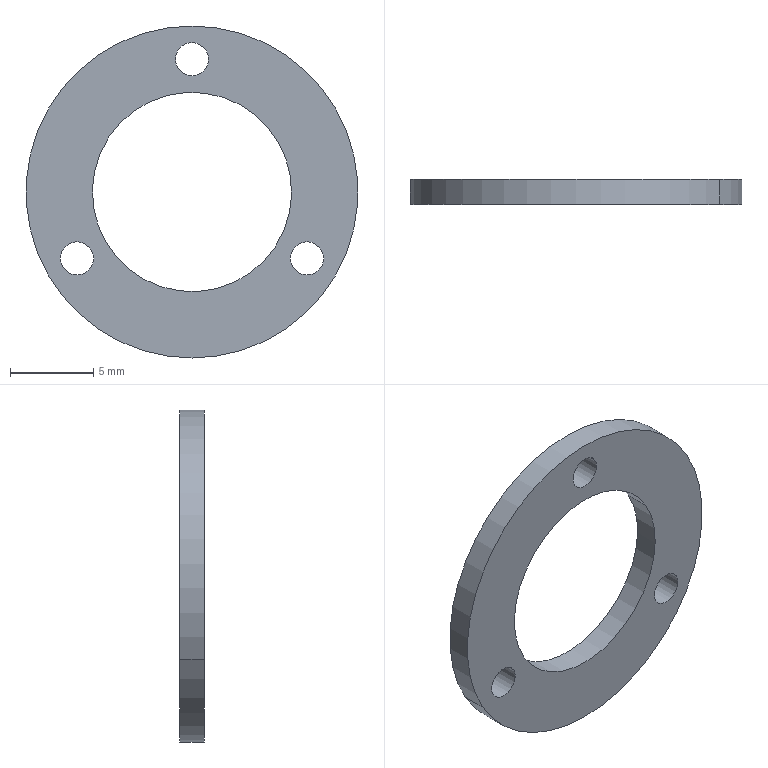Component | SolidWorks | NozzleGasket2-1 | 1 solid | 12 faces | box 20 x 1.5 x 20 mm | volume 287 mm3 | cylinder 10 | plane 2 | commonest cylinder face diameters 2 x6 12 x2 20 x2
build123d program:
from build123d import *

# Parameters (mm, degrees)
SKETCH1_R           = 10
SKETCH1_R_2         = 1
SKETCH1_R_3         = 6
BOSS_EXTRUDE1_DEPTH = 1.5


with BuildPart() as part:
    # Sketch1 → Boss-Extrude1 (new body)
    with BuildSketch(Plane(origin=(0, 0, 0), x_dir=(1, 0, 0), z_dir=(0, 1, 0))):
        with Locations(Location((0, 0, 0), (0, 0, 270))):
            Circle(SKETCH1_R)
        with Locations(Location((0, 8, 0), (0, 0, 270))):
            Circle(SKETCH1_R_2, mode=Mode.SUBTRACT)
        with Locations(Location((6.928, -4, 0), (0, 0, 270))):
            Circle(SKETCH1_R_2, mode=Mode.SUBTRACT)
        with Locations(Location((-6.928, -4, 0), (0, 0, 270))):
            Circle(SKETCH1_R_2, mode=Mode.SUBTRACT)
        with Locations(Location((0, 0, 0), (0, 0, 270))):
            Circle(SKETCH1_R_3, mode=Mode.SUBTRACT)
    extrude(amount=BOSS_EXTRUDE1_DEPTH)


solid = part.part

# Placed as in the assembly
solid = solid.moved(Location((-5.981, -106.494, 160), (180, 0, 0)))
STEP:
#1=COLOUR_RGB('',0.7922,0.8196,0.9333);
#2=FILL_AREA_STYLE_COLOUR('',#1);
#3=FILL_AREA_STYLE('',(#2));
#4=SURFACE_STYLE_FILL_AREA(#3);
#5=SURFACE_SIDE_STYLE('',(#4));
#6=SURFACE_STYLE_USAGE(.BOTH.,#5);
#7=PRESENTATION_STYLE_ASSIGNMENT((#6));
#8=CARTESIAN_POINT('',(-0.2696,-4.193,6.594));
#9=VERTEX_POINT('',#8);
#10=CARTESIAN_POINT('',(-0.2014,-4.193,6.634));
#11=VERTEX_POINT('',#10);
#12=CARTESIAN_POINT('',(-0.2355,-4.193,6.614));
#13=DIRECTION('',(-0.,1.,0.));
#14=DIRECTION('',(0.866,0.,0.5));
#15=AXIS2_PLACEMENT_3D('',#12,#13,#14);
#16=CIRCLE('',#15,0.03937);
#17=EDGE_CURVE('',#9,#11,#16,.T.);
#18=ORIENTED_EDGE('',*,*,#17,.T.);
#19=CARTESIAN_POINT('',(-0.2014,-4.252,6.634));
#20=VERTEX_POINT('',#19);
#21=CARTESIAN_POINT('',(-0.2014,-4.193,6.634));
#22=DIRECTION('',(0.,-1.,-0.));
#23=VECTOR('',#22,39.37);
#24=LINE('',#21,#23);
#25=EDGE_CURVE('',#11,#20,#24,.T.);
#26=ORIENTED_EDGE('',*,*,#25,.T.);
#27=CARTESIAN_POINT('',(-0.2696,-4.252,6.594));
#28=VERTEX_POINT('',#27);
#29=CARTESIAN_POINT('',(-0.2355,-4.252,6.614));
#30=DIRECTION('',(-0.,1.,0.));
#31=DIRECTION('',(0.866,0.,0.5));
#32=AXIS2_PLACEMENT_3D('',#29,#30,#31);
#33=CIRCLE('',#32,0.03937);
#34=EDGE_CURVE('',#28,#20,#33,.T.);
#35=ORIENTED_EDGE('',*,*,#34,.F.);
#36=CARTESIAN_POINT('',(-0.2696,-4.193,6.594));
#37=DIRECTION('',(0.,-1.,-0.));
#38=VECTOR('',#37,39.37);
#39=LINE('',#36,#38);
#40=EDGE_CURVE('',#9,#28,#39,.T.);
#41=ORIENTED_EDGE('',*,*,#40,.F.);
#42=EDGE_LOOP('',(#18,#26,#35,#41));
#43=FACE_OUTER_BOUND('',#42,.T.);
#44=CARTESIAN_POINT('',(-0.2355,-4.193,6.614));
#45=DIRECTION('',(0.,-1.,-0.));
#46=DIRECTION('',(-0.866,0.,-0.5));
#47=AXIS2_PLACEMENT_3D('',#44,#45,#46);
#48=CYLINDRICAL_SURFACE('',#47,0.03937);
#49=ADVANCED_FACE('',(#43),#48,.F.);
#50=CARTESIAN_POINT('',(0.0032,-4.193,6.122));
#51=VERTEX_POINT('',#50);
#52=CARTESIAN_POINT('',(0.07139,-4.193,6.161));
#53=VERTEX_POINT('',#52);
#54=CARTESIAN_POINT('',(0.0373,-4.193,6.142));
#55=DIRECTION('',(-0.,1.,0.));
#56=DIRECTION('',(0.866,0.,0.5));
#57=AXIS2_PLACEMENT_3D('',#54,#55,#56);
#58=CIRCLE('',#57,0.03937);
#59=EDGE_CURVE('',#51,#53,#58,.T.);
#60=ORIENTED_EDGE('',*,*,#59,.T.);
#61=CARTESIAN_POINT('',(0.07139,-4.252,6.161));
#62=VERTEX_POINT('',#61);
#63=CARTESIAN_POINT('',(0.07139,-4.193,6.161));
#64=DIRECTION('',(0.,-1.,-0.));
#65=VECTOR('',#64,39.37);
#66=LINE('',#63,#65);
#67=EDGE_CURVE('',#53,#62,#66,.T.);
#68=ORIENTED_EDGE('',*,*,#67,.T.);
#69=CARTESIAN_POINT('',(0.0032,-4.252,6.122));
#70=VERTEX_POINT('',#69);
#71=CARTESIAN_POINT('',(0.0373,-4.252,6.142));
#72=DIRECTION('',(-0.,1.,0.));
#73=DIRECTION('',(0.866,0.,0.5));
#74=AXIS2_PLACEMENT_3D('',#71,#72,#73);
#75=CIRCLE('',#74,0.03937);
#76=EDGE_CURVE('',#70,#62,#75,.T.);
#77=ORIENTED_EDGE('',*,*,#76,.F.);
#78=CARTESIAN_POINT('',(0.0032,-4.193,6.122));
#79=DIRECTION('',(0.,-1.,-0.));
#80=VECTOR('',#79,39.37);
#81=LINE('',#78,#80);
#82=EDGE_CURVE('',#51,#70,#81,.T.);
#83=ORIENTED_EDGE('',*,*,#82,.F.);
#84=EDGE_LOOP('',(#60,#68,#77,#83));
#85=FACE_OUTER_BOUND('',#84,.T.);
#86=CARTESIAN_POINT('',(0.0373,-4.193,6.142));
#87=DIRECTION('',(0.,-1.,-0.));
#88=DIRECTION('',(-0.866,0.,-0.5));
#89=AXIS2_PLACEMENT_3D('',#86,#87,#88);
#90=CYLINDRICAL_SURFACE('',#89,0.03937);
#91=ADVANCED_FACE('',(#85),#90,.F.);
#92=CARTESIAN_POINT('',(-0.44,-4.193,6.181));
#93=VERTEX_POINT('',#92);
#94=CARTESIAN_POINT('',(-0.0309,-4.193,6.417));
#95=VERTEX_POINT('',#94);
#96=CARTESIAN_POINT('',(-0.2355,-4.193,6.299));
#97=DIRECTION('',(-0.,1.,0.));
#98=DIRECTION('',(0.866,0.,0.5));
#99=AXIS2_PLACEMENT_3D('',#96,#97,#98);
#100=CIRCLE('',#99,0.2362);
#101=EDGE_CURVE('',#93,#95,#100,.T.);
#102=ORIENTED_EDGE('',*,*,#101,.T.);
#103=CARTESIAN_POINT('',(-0.0309,-4.252,6.417));
#104=VERTEX_POINT('',#103);
#105=CARTESIAN_POINT('',(-0.0309,-4.193,6.417));
#106=DIRECTION('',(0.,-1.,-0.));
#107=VECTOR('',#106,39.37);
#108=LINE('',#105,#107);
#109=EDGE_CURVE('',#95,#104,#108,.T.);
#110=ORIENTED_EDGE('',*,*,#109,.T.);
#111=CARTESIAN_POINT('',(-0.44,-4.252,6.181));
#112=VERTEX_POINT('',#111);
#113=CARTESIAN_POINT('',(-0.2355,-4.252,6.299));
#114=DIRECTION('',(-0.,1.,0.));
#115=DIRECTION('',(0.866,0.,0.5));
#116=AXIS2_PLACEMENT_3D('',#113,#114,#115);
#117=CIRCLE('',#116,0.2362);
#118=EDGE_CURVE('',#112,#104,#117,.T.);
#119=ORIENTED_EDGE('',*,*,#118,.F.);
#120=CARTESIAN_POINT('',(-0.44,-4.193,6.181));
#121=DIRECTION('',(0.,-1.,-0.));
#122=VECTOR('',#121,39.37);
#123=LINE('',#120,#122);
#124=EDGE_CURVE('',#93,#112,#123,.T.);
#125=ORIENTED_EDGE('',*,*,#124,.F.);
#126=EDGE_LOOP('',(#102,#110,#119,#125));
#127=FACE_OUTER_BOUND('',#126,.T.);
#128=CARTESIAN_POINT('',(-0.2355,-4.193,6.299));
#129=DIRECTION('',(0.,-1.,-0.));
#130=DIRECTION('',(-0.866,0.,-0.5));
#131=AXIS2_PLACEMENT_3D('',#128,#129,#130);
#132=CYLINDRICAL_SURFACE('',#131,0.2362);
#133=ADVANCED_FACE('',(#127),#132,.F.);
#134=CARTESIAN_POINT('',(-0.5423,-4.193,6.122));
#135=VERTEX_POINT('',#134);
#136=CARTESIAN_POINT('',(-0.4741,-4.193,6.161));
#137=VERTEX_POINT('',#136);
#138=CARTESIAN_POINT('',(-0.5082,-4.193,6.142));
#139=DIRECTION('',(-0.,1.,0.));
#140=DIRECTION('',(0.866,0.,0.5));
#141=AXIS2_PLACEMENT_3D('',#138,#139,#140);
#142=CIRCLE('',#141,0.03937);
#143=EDGE_CURVE('',#135,#137,#142,.T.);
#144=ORIENTED_EDGE('',*,*,#143,.T.);
#145=CARTESIAN_POINT('',(-0.4741,-4.252,6.161));
#146=VERTEX_POINT('',#145);
#147=CARTESIAN_POINT('',(-0.4741,-4.193,6.161));
#148=DIRECTION('',(0.,-1.,-0.));
#149=VECTOR('',#148,39.37);
#150=LINE('',#147,#149);
#151=EDGE_CURVE('',#137,#146,#150,.T.);
#152=ORIENTED_EDGE('',*,*,#151,.T.);
#153=CARTESIAN_POINT('',(-0.5423,-4.252,6.122));
#154=VERTEX_POINT('',#153);
#155=CARTESIAN_POINT('',(-0.5082,-4.252,6.142));
#156=DIRECTION('',(-0.,1.,0.));
#157=DIRECTION('',(0.866,0.,0.5));
#158=AXIS2_PLACEMENT_3D('',#155,#156,#157);
#159=CIRCLE('',#158,0.03937);
#160=EDGE_CURVE('',#154,#146,#159,.T.);
#161=ORIENTED_EDGE('',*,*,#160,.F.);
#162=CARTESIAN_POINT('',(-0.5423,-4.193,6.122));
#163=DIRECTION('',(0.,-1.,-0.));
#164=VECTOR('',#163,39.37);
#165=LINE('',#162,#164);
#166=EDGE_CURVE('',#135,#154,#165,.T.);
#167=ORIENTED_EDGE('',*,*,#166,.F.);
#168=EDGE_LOOP('',(#144,#152,#161,#167));
#169=FACE_OUTER_BOUND('',#168,.T.);
#170=CARTESIAN_POINT('',(-0.5082,-4.193,6.142));
#171=DIRECTION('',(0.,-1.,-0.));
#172=DIRECTION('',(-0.866,0.,-0.5));
#173=AXIS2_PLACEMENT_3D('',#170,#171,#172);
#174=CYLINDRICAL_SURFACE('',#173,0.03937);
#175=ADVANCED_FACE('',(#169),#174,.F.);
#176=CARTESIAN_POINT('',(0.1055,-4.193,6.496));
#177=VERTEX_POINT('',#176);
#178=CARTESIAN_POINT('',(-0.5764,-4.193,6.102));
#179=VERTEX_POINT('',#178);
#180=CARTESIAN_POINT('',(-0.2355,-4.193,6.299));
#181=DIRECTION('',(-0.,1.,0.));
#182=DIRECTION('',(0.866,0.,0.5));
#183=AXIS2_PLACEMENT_3D('',#180,#181,#182);
#184=CIRCLE('',#183,0.3937);
#185=EDGE_CURVE('',#177,#179,#184,.T.);
#186=ORIENTED_EDGE('',*,*,#185,.F.);
#187=CARTESIAN_POINT('',(0.1055,-4.252,6.496));
#188=VERTEX_POINT('',#187);
#189=CARTESIAN_POINT('',(0.1055,-4.193,6.496));
#190=DIRECTION('',(0.,-1.,-0.));
#191=VECTOR('',#190,39.37);
#192=LINE('',#189,#191);
#193=EDGE_CURVE('',#177,#188,#192,.T.);
#194=ORIENTED_EDGE('',*,*,#193,.T.);
#195=CARTESIAN_POINT('',(-0.5764,-4.252,6.102));
#196=VERTEX_POINT('',#195);
#197=CARTESIAN_POINT('',(-0.2355,-4.252,6.299));
#198=DIRECTION('',(-0.,1.,0.));
#199=DIRECTION('',(0.866,0.,0.5));
#200=AXIS2_PLACEMENT_3D('',#197,#198,#199);
#201=CIRCLE('',#200,0.3937);
#202=EDGE_CURVE('',#188,#196,#201,.T.);
#203=ORIENTED_EDGE('',*,*,#202,.T.);
#204=CARTESIAN_POINT('',(-0.5764,-4.193,6.102));
#205=DIRECTION('',(0.,-1.,-0.));
#206=VECTOR('',#205,39.37);
#207=LINE('',#204,#206);
#208=EDGE_CURVE('',#179,#196,#207,.T.);
#209=ORIENTED_EDGE('',*,*,#208,.F.);
#210=EDGE_LOOP('',(#186,#194,#203,#209));
#211=FACE_OUTER_BOUND('',#210,.T.);
#212=CARTESIAN_POINT('',(-0.2355,-4.193,6.299));
#213=DIRECTION('',(0.,-1.,-0.));
#214=DIRECTION('',(-0.866,0.,-0.5));
#215=AXIS2_PLACEMENT_3D('',#212,#213,#214);
#216=CYLINDRICAL_SURFACE('',#215,0.3937);
#217=ADVANCED_FACE('',(#211),#216,.T.);
#218=ORIENTED_EDGE('',*,*,#59,.F.);
#219=CARTESIAN_POINT('',(0.0373,-4.193,6.142));
#220=DIRECTION('',(-0.,1.,0.));
#221=DIRECTION('',(0.866,0.,0.5));
#222=AXIS2_PLACEMENT_3D('',#219,#220,#221);
#223=CIRCLE('',#222,0.03937);
#224=EDGE_CURVE('',#53,#51,#223,.T.);
#225=ORIENTED_EDGE('',*,*,#224,.F.);
#226=EDGE_LOOP('',(#218,#225));
#227=FACE_BOUND('',#226,.T.);
#228=ORIENTED_EDGE('',*,*,#143,.F.);
#229=CARTESIAN_POINT('',(-0.5082,-4.193,6.142));
#230=DIRECTION('',(-0.,1.,0.));
#231=DIRECTION('',(0.866,0.,0.5));
#232=AXIS2_PLACEMENT_3D('',#229,#230,#231);
#233=CIRCLE('',#232,0.03937);
#234=EDGE_CURVE('',#137,#135,#233,.T.);
#235=ORIENTED_EDGE('',*,*,#234,.F.);
#236=EDGE_LOOP('',(#228,#235));
#237=FACE_BOUND('',#236,.T.);
#238=CARTESIAN_POINT('',(-0.2355,-4.193,6.299));
#239=DIRECTION('',(-0.,1.,0.));
#240=DIRECTION('',(0.866,0.,0.5));
#241=AXIS2_PLACEMENT_3D('',#238,#239,#240);
#242=CIRCLE('',#241,0.3937);
#243=EDGE_CURVE('',#179,#177,#242,.T.);
#244=ORIENTED_EDGE('',*,*,#243,.T.);
#245=ORIENTED_EDGE('',*,*,#185,.T.);
#246=EDGE_LOOP('',(#244,#245));
#247=FACE_OUTER_BOUND('',#246,.T.);
#248=ORIENTED_EDGE('',*,*,#101,.F.);
#249=CARTESIAN_POINT('',(-0.2355,-4.193,6.299));
#250=DIRECTION('',(-0.,1.,0.));
#251=DIRECTION('',(0.866,0.,0.5));
#252=AXIS2_PLACEMENT_3D('',#249,#250,#251);
#253=CIRCLE('',#252,0.2362);
#254=EDGE_CURVE('',#95,#93,#253,.T.);
#255=ORIENTED_EDGE('',*,*,#254,.F.);
#256=EDGE_LOOP('',(#248,#255));
#257=FACE_BOUND('',#256,.T.);
#258=ORIENTED_EDGE('',*,*,#17,.F.);
#259=CARTESIAN_POINT('',(-0.2355,-4.193,6.614));
#260=DIRECTION('',(-0.,1.,0.));
#261=DIRECTION('',(0.866,0.,0.5));
#262=AXIS2_PLACEMENT_3D('',#259,#260,#261);
#263=CIRCLE('',#262,0.03937);
#264=EDGE_CURVE('',#11,#9,#263,.T.);
#265=ORIENTED_EDGE('',*,*,#264,.F.);
#266=EDGE_LOOP('',(#258,#265));
#267=FACE_BOUND('',#266,.T.);
#268=CARTESIAN_POINT('',(-0.2355,-4.193,6.299));
#269=DIRECTION('',(-0.,1.,0.));
#270=DIRECTION('',(0.866,0.,0.5));
#271=AXIS2_PLACEMENT_3D('',#268,#269,#270);
#272=PLANE('',#271);
#273=ADVANCED_FACE('',(#227,#237,#247,#257,#267),#272,.T.);
#274=CARTESIAN_POINT('',(-0.2355,-4.252,6.299));
#275=DIRECTION('',(-0.,1.,0.));
#276=DIRECTION('',(0.866,0.,0.5));
#277=AXIS2_PLACEMENT_3D('',#274,#275,#276);
#278=CIRCLE('',#277,0.3937);
#279=EDGE_CURVE('',#196,#188,#278,.T.);
#280=ORIENTED_EDGE('',*,*,#279,.F.);
#281=ORIENTED_EDGE('',*,*,#202,.F.);
#282=EDGE_LOOP('',(#280,#281));
#283=FACE_OUTER_BOUND('',#282,.T.);
#284=ORIENTED_EDGE('',*,*,#160,.T.);
#285=CARTESIAN_POINT('',(-0.5082,-4.252,6.142));
#286=DIRECTION('',(-0.,1.,0.));
#287=DIRECTION('',(0.866,0.,0.5));
#288=AXIS2_PLACEMENT_3D('',#285,#286,#287);
#289=CIRCLE('',#288,0.03937);
#290=EDGE_CURVE('',#146,#154,#289,.T.);
#291=ORIENTED_EDGE('',*,*,#290,.T.);
#292=EDGE_LOOP('',(#284,#291));
#293=FACE_BOUND('',#292,.T.);
#294=ORIENTED_EDGE('',*,*,#118,.T.);
#295=CARTESIAN_POINT('',(-0.2355,-4.252,6.299));
#296=DIRECTION('',(-0.,1.,0.));
#297=DIRECTION('',(0.866,0.,0.5));
#298=AXIS2_PLACEMENT_3D('',#295,#296,#297);
#299=CIRCLE('',#298,0.2362);
#300=EDGE_CURVE('',#104,#112,#299,.T.);
#301=ORIENTED_EDGE('',*,*,#300,.T.);
#302=EDGE_LOOP('',(#294,#301));
#303=FACE_BOUND('',#302,.T.);
#304=ORIENTED_EDGE('',*,*,#76,.T.);
#305=CARTESIAN_POINT('',(0.0373,-4.252,6.142));
#306=DIRECTION('',(-0.,1.,0.));
#307=DIRECTION('',(0.866,0.,0.5));
#308=AXIS2_PLACEMENT_3D('',#305,#306,#307);
#309=CIRCLE('',#308,0.03937);
#310=EDGE_CURVE('',#62,#70,#309,.T.);
#311=ORIENTED_EDGE('',*,*,#310,.T.);
#312=EDGE_LOOP('',(#304,#311));
#313=FACE_BOUND('',#312,.T.);
#314=ORIENTED_EDGE('',*,*,#34,.T.);
#315=CARTESIAN_POINT('',(-0.2355,-4.252,6.614));
#316=DIRECTION('',(-0.,1.,0.));
#317=DIRECTION('',(0.866,0.,0.5));
#318=AXIS2_PLACEMENT_3D('',#315,#316,#317);
#319=CIRCLE('',#318,0.03937);
#320=EDGE_CURVE('',#20,#28,#319,.T.);
#321=ORIENTED_EDGE('',*,*,#320,.T.);
#322=EDGE_LOOP('',(#314,#321));
#323=FACE_BOUND('',#322,.T.);
#324=CARTESIAN_POINT('',(-0.2355,-4.252,6.299));
#325=DIRECTION('',(-0.,1.,0.));
#326=DIRECTION('',(0.866,0.,0.5));
#327=AXIS2_PLACEMENT_3D('',#324,#325,#326);
#328=PLANE('',#327);
#329=ADVANCED_FACE('',(#283,#293,#303,#313,#323),#328,.F.);
#330=ORIENTED_EDGE('',*,*,#193,.F.);
#331=ORIENTED_EDGE('',*,*,#243,.F.);
#332=ORIENTED_EDGE('',*,*,#208,.T.);
#333=ORIENTED_EDGE('',*,*,#279,.T.);
#334=EDGE_LOOP('',(#330,#331,#332,#333));
#335=FACE_OUTER_BOUND('',#334,.T.);
#336=CARTESIAN_POINT('',(-0.2355,-4.193,6.299));
#337=DIRECTION('',(0.,-1.,-0.));
#338=DIRECTION('',(-0.866,0.,-0.5));
#339=AXIS2_PLACEMENT_3D('',#336,#337,#338);
#340=CYLINDRICAL_SURFACE('',#339,0.3937);
#341=ADVANCED_FACE('',(#335),#340,.T.);
#342=ORIENTED_EDGE('',*,*,#151,.F.);
#343=ORIENTED_EDGE('',*,*,#234,.T.);
#344=ORIENTED_EDGE('',*,*,#166,.T.);
#345=ORIENTED_EDGE('',*,*,#290,.F.);
#346=EDGE_LOOP('',(#342,#343,#344,#345));
#347=FACE_OUTER_BOUND('',#346,.T.);
#348=CARTESIAN_POINT('',(-0.5082,-4.193,6.142));
#349=DIRECTION('',(0.,-1.,-0.));
#350=DIRECTION('',(-0.866,0.,-0.5));
#351=AXIS2_PLACEMENT_3D('',#348,#349,#350);
#352=CYLINDRICAL_SURFACE('',#351,0.03937);
#353=ADVANCED_FACE('',(#347),#352,.F.);
#354=ORIENTED_EDGE('',*,*,#109,.F.);
#355=ORIENTED_EDGE('',*,*,#254,.T.);
#356=ORIENTED_EDGE('',*,*,#124,.T.);
#357=ORIENTED_EDGE('',*,*,#300,.F.);
#358=EDGE_LOOP('',(#354,#355,#356,#357));
#359=FACE_OUTER_BOUND('',#358,.T.);
#360=CARTESIAN_POINT('',(-0.2355,-4.193,6.299));
#361=DIRECTION('',(0.,-1.,-0.));
#362=DIRECTION('',(-0.866,0.,-0.5));
#363=AXIS2_PLACEMENT_3D('',#360,#361,#362);
#364=CYLINDRICAL_SURFACE('',#363,0.2362);
#365=ADVANCED_FACE('',(#359),#364,.F.);
#366=ORIENTED_EDGE('',*,*,#67,.F.);
#367=ORIENTED_EDGE('',*,*,#224,.T.);
#368=ORIENTED_EDGE('',*,*,#82,.T.);
#369=ORIENTED_EDGE('',*,*,#310,.F.);
#370=EDGE_LOOP('',(#366,#367,#368,#369));
#371=FACE_OUTER_BOUND('',#370,.T.);
#372=CARTESIAN_POINT('',(0.0373,-4.193,6.142));
#373=DIRECTION('',(0.,-1.,-0.));
#374=DIRECTION('',(-0.866,0.,-0.5));
#375=AXIS2_PLACEMENT_3D('',#372,#373,#374);
#376=CYLINDRICAL_SURFACE('',#375,0.03937);
#377=ADVANCED_FACE('',(#371),#376,.F.);
#378=ORIENTED_EDGE('',*,*,#25,.F.);
#379=ORIENTED_EDGE('',*,*,#264,.T.);
#380=ORIENTED_EDGE('',*,*,#40,.T.);
#381=ORIENTED_EDGE('',*,*,#320,.F.);
#382=EDGE_LOOP('',(#378,#379,#380,#381));
#383=FACE_OUTER_BOUND('',#382,.T.);
#384=CARTESIAN_POINT('',(-0.2355,-4.193,6.614));
#385=DIRECTION('',(0.,-1.,-0.));
#386=DIRECTION('',(-0.866,0.,-0.5));
#387=AXIS2_PLACEMENT_3D('',#384,#385,#386);
#388=CYLINDRICAL_SURFACE('',#387,0.03937);
#389=ADVANCED_FACE('',(#383),#388,.F.);
#390=CLOSED_SHELL('',(#49,#91,#133,#175,#217,#273,#329,#341,#353,#365,#377,#389));
#391=MANIFOLD_SOLID_BREP('',#390);
#392=STYLED_ITEM('',(#7),#391);
#393=PRESENTATION_LAYER_ASSIGNMENT('','',(#392));
#394=(LENGTH_UNIT()NAMED_UNIT(*)SI_UNIT($,.METRE.));
#395=LENGTH_MEASURE_WITH_UNIT(LENGTH_MEASURE(0.0254),#394);
#396=DIMENSIONAL_EXPONENTS(1.,0.,0.,0.,0.,0.,0.);
#397=(CONVERSION_BASED_UNIT('',#395)LENGTH_UNIT()NAMED_UNIT(#396));
#398=UNCERTAINTY_MEASURE_WITH_UNIT(LENGTH_MEASURE(0.00001),#397,'','');
#399=(NAMED_UNIT(*)PLANE_ANGLE_UNIT()SI_UNIT($,.RADIAN.));
#400=(NAMED_UNIT(*)SI_UNIT($,.STERADIAN.)SOLID_ANGLE_UNIT());
#401=(GEOMETRIC_REPRESENTATION_CONTEXT(3)GLOBAL_UNCERTAINTY_ASSIGNED_CONTEXT((#398))GLOBAL_UNIT_ASSIGNED_CONTEXT((#397,#399,#400))REPRESENTATION_CONTEXT('',''));
#402=MECHANICAL_DESIGN_GEOMETRIC_PRESENTATION_REPRESENTATION('',(#392),#401);
#403=CARTESIAN_POINT('',(0.,0.,0.));
#404=DIRECTION('',(0.,0.,1.));
#405=DIRECTION('',(1.,0.,0.));
#406=AXIS2_PLACEMENT_3D('',#403,#404,#405);
#407=(LENGTH_UNIT()NAMED_UNIT(*)SI_UNIT($,.METRE.));
#408=LENGTH_MEASURE_WITH_UNIT(LENGTH_MEASURE(0.0254),#407);
#409=DIMENSIONAL_EXPONENTS(1.,0.,0.,0.,0.,0.,0.);
#410=(CONVERSION_BASED_UNIT('',#408)LENGTH_UNIT()NAMED_UNIT(#409));
#411=UNCERTAINTY_MEASURE_WITH_UNIT(LENGTH_MEASURE(0.00001),#410,'','');
#412=(NAMED_UNIT(*)PLANE_ANGLE_UNIT()SI_UNIT($,.RADIAN.));
#413=(NAMED_UNIT(*)SI_UNIT($,.STERADIAN.)SOLID_ANGLE_UNIT());
#414=(GEOMETRIC_REPRESENTATION_CONTEXT(3)GLOBAL_UNCERTAINTY_ASSIGNED_CONTEXT((#411))GLOBAL_UNIT_ASSIGNED_CONTEXT((#410,#412,#413))REPRESENTATION_CONTEXT('',''));
#415=ADVANCED_BREP_SHAPE_REPRESENTATION('',(#391,#406),#414);